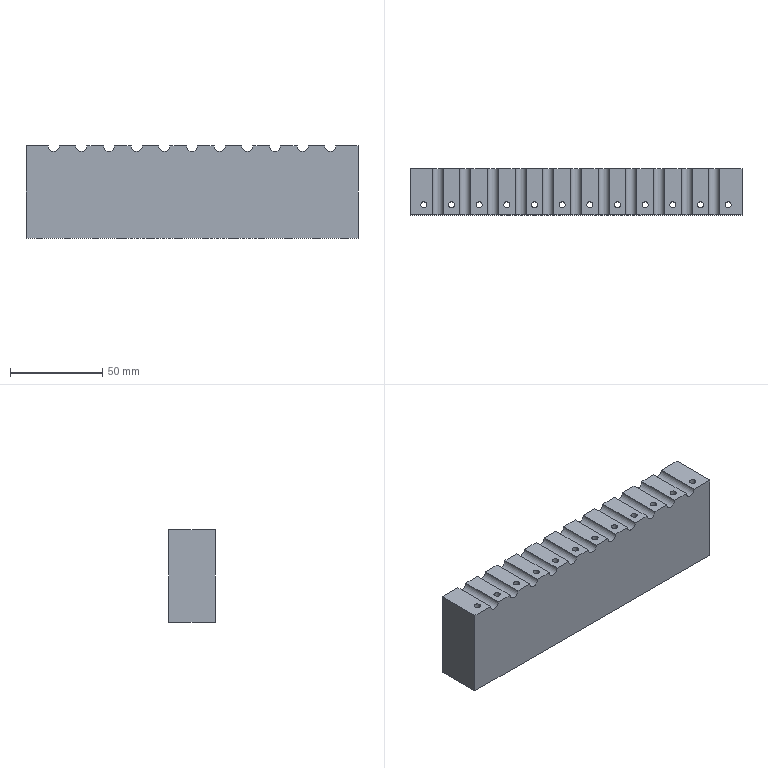CAM job | Mastercam | mm | 10 operations | part box 180 x 25 x 50
1. Drill/Counterbore | 7 - 4 倒角刀
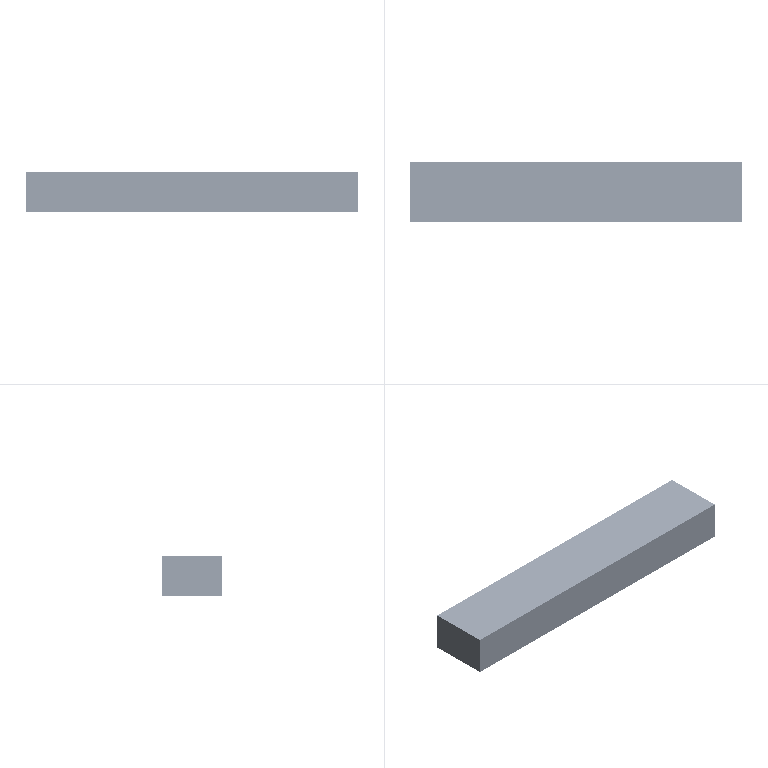2. Peck Drill | 1 - 3.3 钻头
3. Contour (2D chamfer) | 7 - 4 倒角刀
4. Tap | 2 - M4 x 0.7 右牙
5. Contour (Ramp) | 5 - 6 球刀/圆鼻铣刀
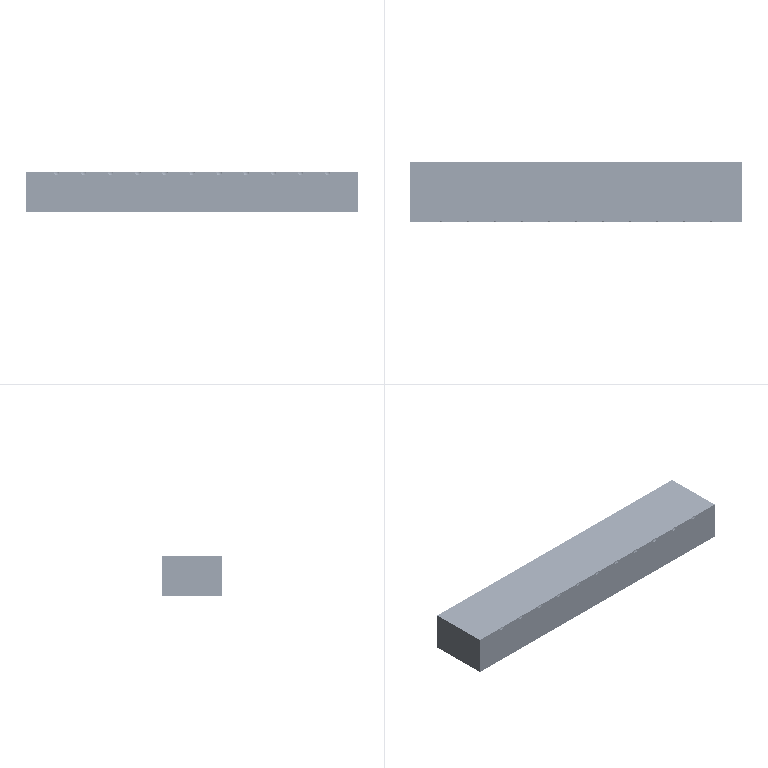6. Contour (2D) | 5 - 6 球刀/圆鼻铣刀
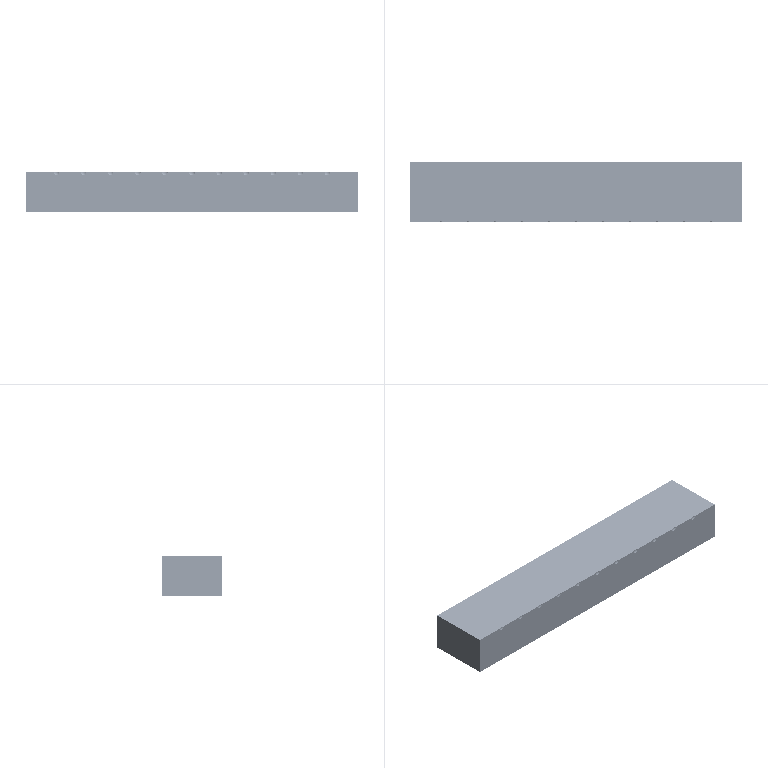7. Deburr 5-axis | 5 - 6 球刀/圆鼻铣刀
8. Drill/Counterbore | 7 - 4 倒角刀
9. Peck Drill | 3 - 4 钻头
10. Contour (2D chamfer) | 7 - 4 倒角刀